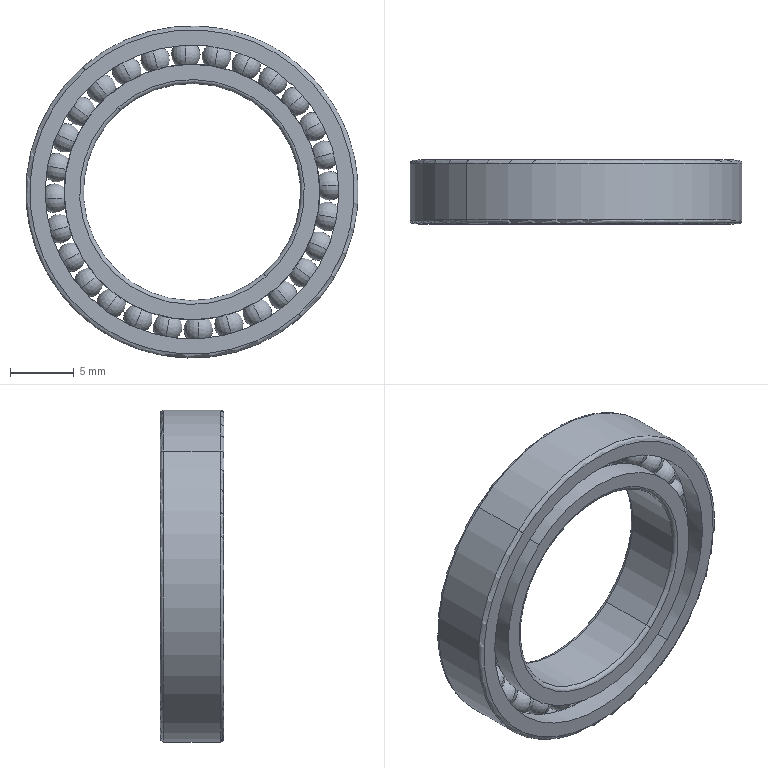Component | SolidWorks | CrankshaftOne-1_deep groove ball bearings gb-1 | 1 solid | 164 faces | volume 1118 mm3 | torus 92 | sphere 56 | cylinder 12 | plane 4 | commonest cylinder face diameters 23 x4 20 x4 26 x2 17 x2